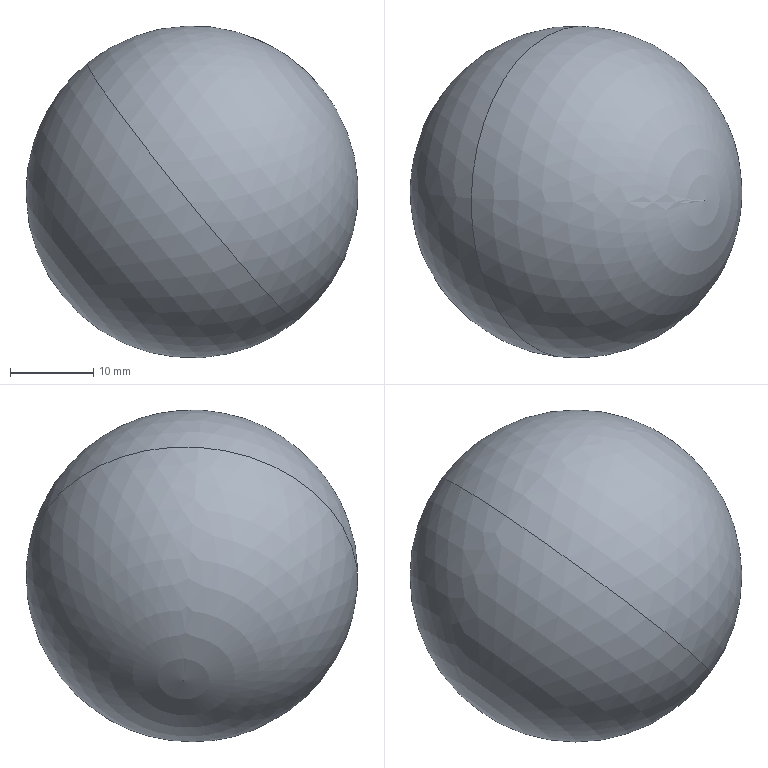Component | SolidWorks | ClampingMechanism-1_BallJoint-1 | 1 solid | 2 faces | box 40 x 40 x 40 mm | volume 33510 mm3 | sphere 2
build123d program:
from build123d import *


with BuildPart() as part:
    # Sketch1 → Revolve1 (revolve)
    with BuildSketch(Plane.XY):
        with BuildLine():
            Line((0, 20), (0, -20))
            ThreePointArc((0, -20), (20, 0), (0, 20))
        make_face()
    revolve(axis=Axis((0, 20, 0), (0, -1, 0)))


solid = part.part

# Placed as in the assembly
solid = solid.moved(Location((69.427, -208.758, -542.97), (0, 0, 0)))
STEP:
#1=COLOUR_RGB('',0.7922,0.8196,0.9333);
#2=FILL_AREA_STYLE_COLOUR('',#1);
#3=FILL_AREA_STYLE('',(#2));
#4=SURFACE_STYLE_FILL_AREA(#3);
#5=SURFACE_SIDE_STYLE('',(#4));
#6=SURFACE_STYLE_USAGE(.BOTH.,#5);
#7=PRESENTATION_STYLE_ASSIGNMENT((#6));
#8=CARTESIAN_POINT('',(2.72,-9.005,-21.426));
#9=VERTEX_POINT('',#8);
#10=CARTESIAN_POINT('',(2.746,-7.433,-21.327));
#11=VERTEX_POINT('',#10);
#12=CARTESIAN_POINT('',(2.733,-8.219,-21.377));
#13=DIRECTION('',(-0.7752,0.05261,-0.6296));
#14=DIRECTION('',(-0.6305,0.,0.7762));
#15=AXIS2_PLACEMENT_3D('',#12,#13,#14);
#16=CIRCLE('',#15,0.7874);
#17=EDGE_CURVE('',#9,#11,#16,.T.);
#18=ORIENTED_EDGE('',*,*,#17,.F.);
#19=CARTESIAN_POINT('',(2.733,-8.219,-21.377));
#20=DIRECTION('',(0.7752,-0.05261,0.6296));
#21=DIRECTION('',(0.6305,0.,-0.7762));
#22=AXIS2_PLACEMENT_3D('',#19,#20,#21);
#23=CIRCLE('',#22,0.7874);
#24=EDGE_CURVE('',#9,#11,#23,.T.);
#25=ORIENTED_EDGE('',*,*,#24,.T.);
#26=EDGE_LOOP('',(#18,#25));
#27=FACE_OUTER_BOUND('',#26,.T.);
#28=CARTESIAN_POINT('',(2.733,-8.219,-21.377));
#29=DIRECTION('',(0.7752,-0.05261,0.6296));
#30=DIRECTION('',(-0.6316,-0.03835,0.7744));
#31=AXIS2_PLACEMENT_3D('',#28,#29,#30);
#32=SPHERICAL_SURFACE('',#31,0.7874);
#33=ADVANCED_FACE('',(#27),#32,.T.);
#34=ORIENTED_EDGE('',*,*,#24,.F.);
#35=ORIENTED_EDGE('',*,*,#17,.T.);
#36=EDGE_LOOP('',(#34,#35));
#37=FACE_OUTER_BOUND('',#36,.T.);
#38=CARTESIAN_POINT('',(2.733,-8.219,-21.377));
#39=DIRECTION('',(0.7752,-0.05261,0.6296));
#40=DIRECTION('',(-0.6316,-0.03835,0.7744));
#41=AXIS2_PLACEMENT_3D('',#38,#39,#40);
#42=SPHERICAL_SURFACE('',#41,0.7874);
#43=ADVANCED_FACE('',(#37),#42,.T.);
#44=CLOSED_SHELL('',(#33,#43));
#45=MANIFOLD_SOLID_BREP('',#44);
#46=STYLED_ITEM('',(#7),#45);
#47=PRESENTATION_LAYER_ASSIGNMENT('','',(#46));
#48=(LENGTH_UNIT()NAMED_UNIT(*)SI_UNIT($,.METRE.));
#49=LENGTH_MEASURE_WITH_UNIT(LENGTH_MEASURE(0.0254),#48);
#50=DIMENSIONAL_EXPONENTS(1.,0.,0.,0.,0.,0.,0.);
#51=(CONVERSION_BASED_UNIT('',#49)LENGTH_UNIT()NAMED_UNIT(#50));
#52=UNCERTAINTY_MEASURE_WITH_UNIT(LENGTH_MEASURE(0.00001),#51,'','');
#53=(NAMED_UNIT(*)PLANE_ANGLE_UNIT()SI_UNIT($,.RADIAN.));
#54=(NAMED_UNIT(*)SI_UNIT($,.STERADIAN.)SOLID_ANGLE_UNIT());
#55=(GEOMETRIC_REPRESENTATION_CONTEXT(3)GLOBAL_UNCERTAINTY_ASSIGNED_CONTEXT((#52))GLOBAL_UNIT_ASSIGNED_CONTEXT((#51,#53,#54))REPRESENTATION_CONTEXT('',''));
#56=MECHANICAL_DESIGN_GEOMETRIC_PRESENTATION_REPRESENTATION('',(#46),#55);
#57=CARTESIAN_POINT('',(0.,0.,0.));
#58=DIRECTION('',(0.,0.,1.));
#59=DIRECTION('',(1.,0.,0.));
#60=AXIS2_PLACEMENT_3D('',#57,#58,#59);
#61=(LENGTH_UNIT()NAMED_UNIT(*)SI_UNIT($,.METRE.));
#62=LENGTH_MEASURE_WITH_UNIT(LENGTH_MEASURE(0.0254),#61);
#63=DIMENSIONAL_EXPONENTS(1.,0.,0.,0.,0.,0.,0.);
#64=(CONVERSION_BASED_UNIT('',#62)LENGTH_UNIT()NAMED_UNIT(#63));
#65=UNCERTAINTY_MEASURE_WITH_UNIT(LENGTH_MEASURE(0.00001),#64,'','');
#66=(NAMED_UNIT(*)PLANE_ANGLE_UNIT()SI_UNIT($,.RADIAN.));
#67=(NAMED_UNIT(*)SI_UNIT($,.STERADIAN.)SOLID_ANGLE_UNIT());
#68=(GEOMETRIC_REPRESENTATION_CONTEXT(3)GLOBAL_UNCERTAINTY_ASSIGNED_CONTEXT((#65))GLOBAL_UNIT_ASSIGNED_CONTEXT((#64,#66,#67))REPRESENTATION_CONTEXT('',''));
#69=ADVANCED_BREP_SHAPE_REPRESENTATION('',(#45,#60),#68);